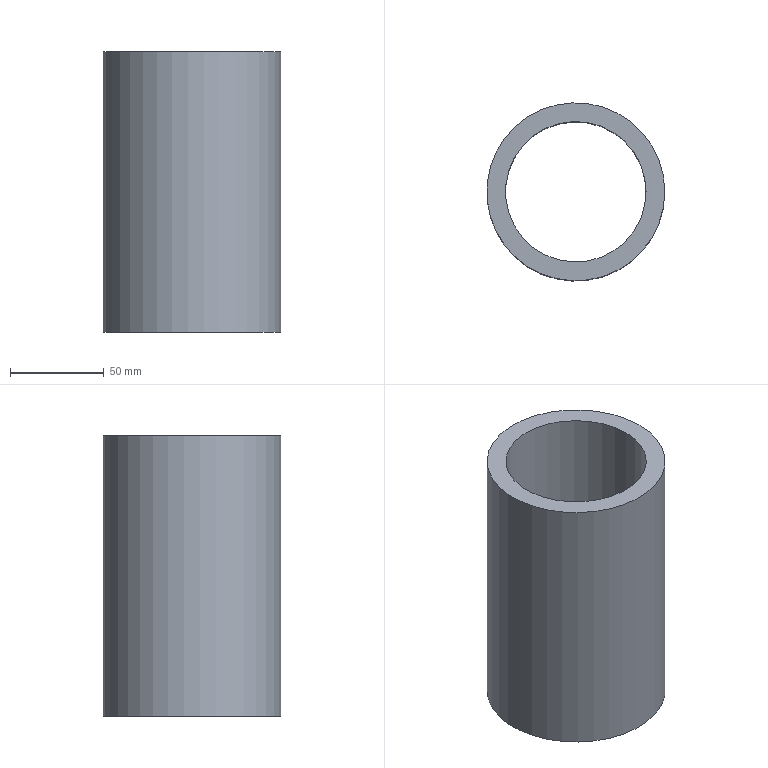Component | NX | CIRCLE | 1 solid | 4 faces | box 95 x 95 x 150 mm | volume 400553 mm3 | cylinder 2 | plane 2 | commonest cylinder face diameters 95 x1 75 x1
STEP:
#1=CARTESIAN_POINT('',(0.,0.,0.));
#2=DIRECTION('',(0.,0.,1.));
#3=DIRECTION('',(1.,0.,0.));
#4=AXIS2_PLACEMENT_3D('',#1,#2,#3);
#5=CARTESIAN_POINT('',(-152.5,20.,170.));
#6=VERTEX_POINT('',#5);
#7=CARTESIAN_POINT('',(-200.,20.,170.));
#8=DIRECTION('',(0.,0.,1.));
#9=DIRECTION('',(1.,0.,0.));
#10=AXIS2_PLACEMENT_3D('',#7,#8,#9);
#11=CIRCLE('',#10,47.5);
#12=CARTESIAN_POINT('',(-200.,20.,170.));
#13=DIRECTION('',(0.,0.,-1.));
#14=DIRECTION('',(-1.,0.,0.));
#15=AXIS2_PLACEMENT_3D('',#12,#13,#14);
#16=CYLINDRICAL_SURFACE('',#15,47.5);
#17=CARTESIAN_POINT('',(9.425,0.));
#18=DIRECTION('',(-1.,0.));
#19=VECTOR('',#18,1.);
#20=LINE('',#17,#19);
#21=(GEOMETRIC_REPRESENTATION_CONTEXT(2)PARAMETRIC_REPRESENTATION_CONTEXT()REPRESENTATION_CONTEXT('',''));
#22=DEFINITIONAL_REPRESENTATION('',(#20),#21);
#23=PCURVE('',#16,#22);
#24=CARTESIAN_POINT('',(-200.,20.,170.));
#25=DIRECTION('',(0.,0.,1.));
#26=DIRECTION('',(1.,0.,0.));
#27=AXIS2_PLACEMENT_3D('',#24,#25,#26);
#28=PLANE('',#27);
#29=CARTESIAN_POINT('',(0.,0.));
#30=DIRECTION('',(1.,0.));
#31=AXIS2_PLACEMENT_2D('',#29,#30);
#32=CIRCLE('',#31,47.5);
#33=(GEOMETRIC_REPRESENTATION_CONTEXT(2)PARAMETRIC_REPRESENTATION_CONTEXT()REPRESENTATION_CONTEXT('',''));
#34=DEFINITIONAL_REPRESENTATION('',(#32),#33);
#35=PCURVE('',#28,#34);
#36=SURFACE_CURVE('',#11,(#23,#35),.PCURVE_S1.);
#37=EDGE_CURVE('',#6,#6,#36,.T.);
#38=ORIENTED_EDGE('',*,*,#37,.F.);
#39=CARTESIAN_POINT('',(-152.5,20.,20.));
#40=VERTEX_POINT('',#39);
#41=CARTESIAN_POINT('',(-152.5,20.,170.));
#42=CARTESIAN_POINT('',(-152.5,20.,20.));
#43=B_SPLINE_CURVE_WITH_KNOTS('',1,(#41,#42),.UNSPECIFIED.,.F.,.F.,(2,2),(0.,150.),.PIECEWISE_BEZIER_KNOTS.);
#44=CARTESIAN_POINT('',(9.425,0.));
#45=DIRECTION('',(0.,1.));
#46=VECTOR('',#45,1.);
#47=LINE('',#44,#46);
#48=(GEOMETRIC_REPRESENTATION_CONTEXT(2)PARAMETRIC_REPRESENTATION_CONTEXT()REPRESENTATION_CONTEXT('',''));
#49=DEFINITIONAL_REPRESENTATION('',(#47),#48);
#50=PCURVE('',#16,#49);
#51=CARTESIAN_POINT('',(3.142,0.));
#52=DIRECTION('',(0.,1.));
#53=VECTOR('',#52,1.);
#54=LINE('',#51,#53);
#55=(GEOMETRIC_REPRESENTATION_CONTEXT(2)PARAMETRIC_REPRESENTATION_CONTEXT()REPRESENTATION_CONTEXT('',''));
#56=DEFINITIONAL_REPRESENTATION('',(#54),#55);
#57=PCURVE('',#16,#56);
#58=SEAM_CURVE('',#43,(#50,#57),.PCURVE_S1.);
#59=EDGE_CURVE('',#6,#40,#58,.T.);
#60=ORIENTED_EDGE('',*,*,#59,.T.);
#61=CARTESIAN_POINT('',(-200.,20.,20.));
#62=DIRECTION('',(0.,0.,1.));
#63=DIRECTION('',(1.,0.,0.));
#64=AXIS2_PLACEMENT_3D('',#61,#62,#63);
#65=CIRCLE('',#64,47.5);
#66=CARTESIAN_POINT('',(9.425,150.));
#67=DIRECTION('',(-1.,0.));
#68=VECTOR('',#67,1.);
#69=LINE('',#66,#68);
#70=(GEOMETRIC_REPRESENTATION_CONTEXT(2)PARAMETRIC_REPRESENTATION_CONTEXT()REPRESENTATION_CONTEXT('',''));
#71=DEFINITIONAL_REPRESENTATION('',(#69),#70);
#72=PCURVE('',#16,#71);
#73=CARTESIAN_POINT('',(-200.,20.,20.));
#74=DIRECTION('',(0.,0.,1.));
#75=DIRECTION('',(1.,0.,0.));
#76=AXIS2_PLACEMENT_3D('',#73,#74,#75);
#77=PLANE('',#76);
#78=CARTESIAN_POINT('',(0.,0.));
#79=DIRECTION('',(1.,0.));
#80=AXIS2_PLACEMENT_2D('',#78,#79);
#81=CIRCLE('',#80,47.5);
#82=(GEOMETRIC_REPRESENTATION_CONTEXT(2)PARAMETRIC_REPRESENTATION_CONTEXT()REPRESENTATION_CONTEXT('',''));
#83=DEFINITIONAL_REPRESENTATION('',(#81),#82);
#84=PCURVE('',#77,#83);
#85=SURFACE_CURVE('',#65,(#72,#84),.PCURVE_S1.);
#86=EDGE_CURVE('',#40,#40,#85,.T.);
#87=ORIENTED_EDGE('',*,*,#86,.T.);
#88=ORIENTED_EDGE('',*,*,#59,.F.);
#89=EDGE_LOOP('',(#38,#60,#87,#88));
#90=FACE_BOUND('',#89,.T.);
#91=ADVANCED_FACE('',(#90),#16,.T.);
#92=CARTESIAN_POINT('',(-162.5,20.,170.));
#93=VERTEX_POINT('',#92);
#94=CARTESIAN_POINT('',(-200.,20.,170.));
#95=DIRECTION('',(0.,0.,1.));
#96=DIRECTION('',(1.,0.,0.));
#97=AXIS2_PLACEMENT_3D('',#94,#95,#96);
#98=CIRCLE('',#97,37.5);
#99=CARTESIAN_POINT('',(-200.,20.,170.));
#100=DIRECTION('',(0.,0.,-1.));
#101=DIRECTION('',(-1.,0.,0.));
#102=AXIS2_PLACEMENT_3D('',#99,#100,#101);
#103=CYLINDRICAL_SURFACE('',#102,37.5);
#104=CARTESIAN_POINT('',(9.425,0.));
#105=DIRECTION('',(-1.,0.));
#106=VECTOR('',#105,1.);
#107=LINE('',#104,#106);
#108=(GEOMETRIC_REPRESENTATION_CONTEXT(2)PARAMETRIC_REPRESENTATION_CONTEXT()REPRESENTATION_CONTEXT('',''));
#109=DEFINITIONAL_REPRESENTATION('',(#107),#108);
#110=PCURVE('',#103,#109);
#111=CARTESIAN_POINT('',(0.,0.));
#112=DIRECTION('',(1.,0.));
#113=AXIS2_PLACEMENT_2D('',#111,#112);
#114=CIRCLE('',#113,37.5);
#115=(GEOMETRIC_REPRESENTATION_CONTEXT(2)PARAMETRIC_REPRESENTATION_CONTEXT()REPRESENTATION_CONTEXT('',''));
#116=DEFINITIONAL_REPRESENTATION('',(#114),#115);
#117=PCURVE('',#28,#116);
#118=SURFACE_CURVE('',#98,(#110,#117),.PCURVE_S1.);
#119=EDGE_CURVE('',#93,#93,#118,.T.);
#120=ORIENTED_EDGE('',*,*,#119,.F.);
#121=CARTESIAN_POINT('',(-162.5,20.,20.));
#122=VERTEX_POINT('',#121);
#123=CARTESIAN_POINT('',(-162.5,20.,170.));
#124=CARTESIAN_POINT('',(-162.5,20.,20.));
#125=B_SPLINE_CURVE_WITH_KNOTS('',1,(#123,#124),.UNSPECIFIED.,.F.,.F.,(2,2),(0.,150.),.PIECEWISE_BEZIER_KNOTS.);
#126=CARTESIAN_POINT('',(9.425,0.));
#127=DIRECTION('',(0.,1.));
#128=VECTOR('',#127,1.);
#129=LINE('',#126,#128);
#130=(GEOMETRIC_REPRESENTATION_CONTEXT(2)PARAMETRIC_REPRESENTATION_CONTEXT()REPRESENTATION_CONTEXT('',''));
#131=DEFINITIONAL_REPRESENTATION('',(#129),#130);
#132=PCURVE('',#103,#131);
#133=CARTESIAN_POINT('',(3.142,0.));
#134=DIRECTION('',(0.,1.));
#135=VECTOR('',#134,1.);
#136=LINE('',#133,#135);
#137=(GEOMETRIC_REPRESENTATION_CONTEXT(2)PARAMETRIC_REPRESENTATION_CONTEXT()REPRESENTATION_CONTEXT('',''));
#138=DEFINITIONAL_REPRESENTATION('',(#136),#137);
#139=PCURVE('',#103,#138);
#140=SEAM_CURVE('',#125,(#132,#139),.PCURVE_S1.);
#141=EDGE_CURVE('',#93,#122,#140,.T.);
#142=ORIENTED_EDGE('',*,*,#141,.T.);
#143=CARTESIAN_POINT('',(-200.,20.,20.));
#144=DIRECTION('',(0.,0.,1.));
#145=DIRECTION('',(1.,0.,0.));
#146=AXIS2_PLACEMENT_3D('',#143,#144,#145);
#147=CIRCLE('',#146,37.5);
#148=CARTESIAN_POINT('',(9.425,150.));
#149=DIRECTION('',(-1.,0.));
#150=VECTOR('',#149,1.);
#151=LINE('',#148,#150);
#152=(GEOMETRIC_REPRESENTATION_CONTEXT(2)PARAMETRIC_REPRESENTATION_CONTEXT()REPRESENTATION_CONTEXT('',''));
#153=DEFINITIONAL_REPRESENTATION('',(#151),#152);
#154=PCURVE('',#103,#153);
#155=CARTESIAN_POINT('',(0.,0.));
#156=DIRECTION('',(1.,0.));
#157=AXIS2_PLACEMENT_2D('',#155,#156);
#158=CIRCLE('',#157,37.5);
#159=(GEOMETRIC_REPRESENTATION_CONTEXT(2)PARAMETRIC_REPRESENTATION_CONTEXT()REPRESENTATION_CONTEXT('',''));
#160=DEFINITIONAL_REPRESENTATION('',(#158),#159);
#161=PCURVE('',#77,#160);
#162=SURFACE_CURVE('',#147,(#154,#161),.PCURVE_S1.);
#163=EDGE_CURVE('',#122,#122,#162,.T.);
#164=ORIENTED_EDGE('',*,*,#163,.T.);
#165=ORIENTED_EDGE('',*,*,#141,.F.);
#166=EDGE_LOOP('',(#120,#142,#164,#165));
#167=FACE_BOUND('',#166,.F.);
#168=ADVANCED_FACE('',(#167),#103,.F.);
#169=ORIENTED_EDGE('',*,*,#37,.T.);
#170=EDGE_LOOP('',(#169));
#171=FACE_BOUND('',#170,.T.);
#172=ORIENTED_EDGE('',*,*,#119,.F.);
#173=EDGE_LOOP('',(#172));
#174=FACE_BOUND('',#173,.T.);
#175=ADVANCED_FACE('',(#171,#174),#28,.T.);
#176=ORIENTED_EDGE('',*,*,#86,.F.);
#177=EDGE_LOOP('',(#176));
#178=FACE_BOUND('',#177,.T.);
#179=ORIENTED_EDGE('',*,*,#163,.T.);
#180=EDGE_LOOP('',(#179));
#181=FACE_BOUND('',#180,.T.);
#182=ADVANCED_FACE('',(#178,#181),#77,.F.);
#183=CLOSED_SHELL('',(#91,#168,#175,#182));
#184=MANIFOLD_SOLID_BREP('',#183);
#185=(LENGTH_UNIT()NAMED_UNIT(*)SI_UNIT(.MILLI.,.METRE.));
#186=UNCERTAINTY_MEASURE_WITH_UNIT(LENGTH_MEASURE(0.00001),#185,'','');
#187=(NAMED_UNIT(*)PLANE_ANGLE_UNIT()SI_UNIT($,.RADIAN.));
#188=(NAMED_UNIT(*)SI_UNIT($,.STERADIAN.)SOLID_ANGLE_UNIT());
#189=(GEOMETRIC_REPRESENTATION_CONTEXT(3)GLOBAL_UNCERTAINTY_ASSIGNED_CONTEXT((#186))GLOBAL_UNIT_ASSIGNED_CONTEXT((#185,#187,#188))REPRESENTATION_CONTEXT('',''));
#190=ADVANCED_BREP_SHAPE_REPRESENTATION('',(#4,#184),#189);